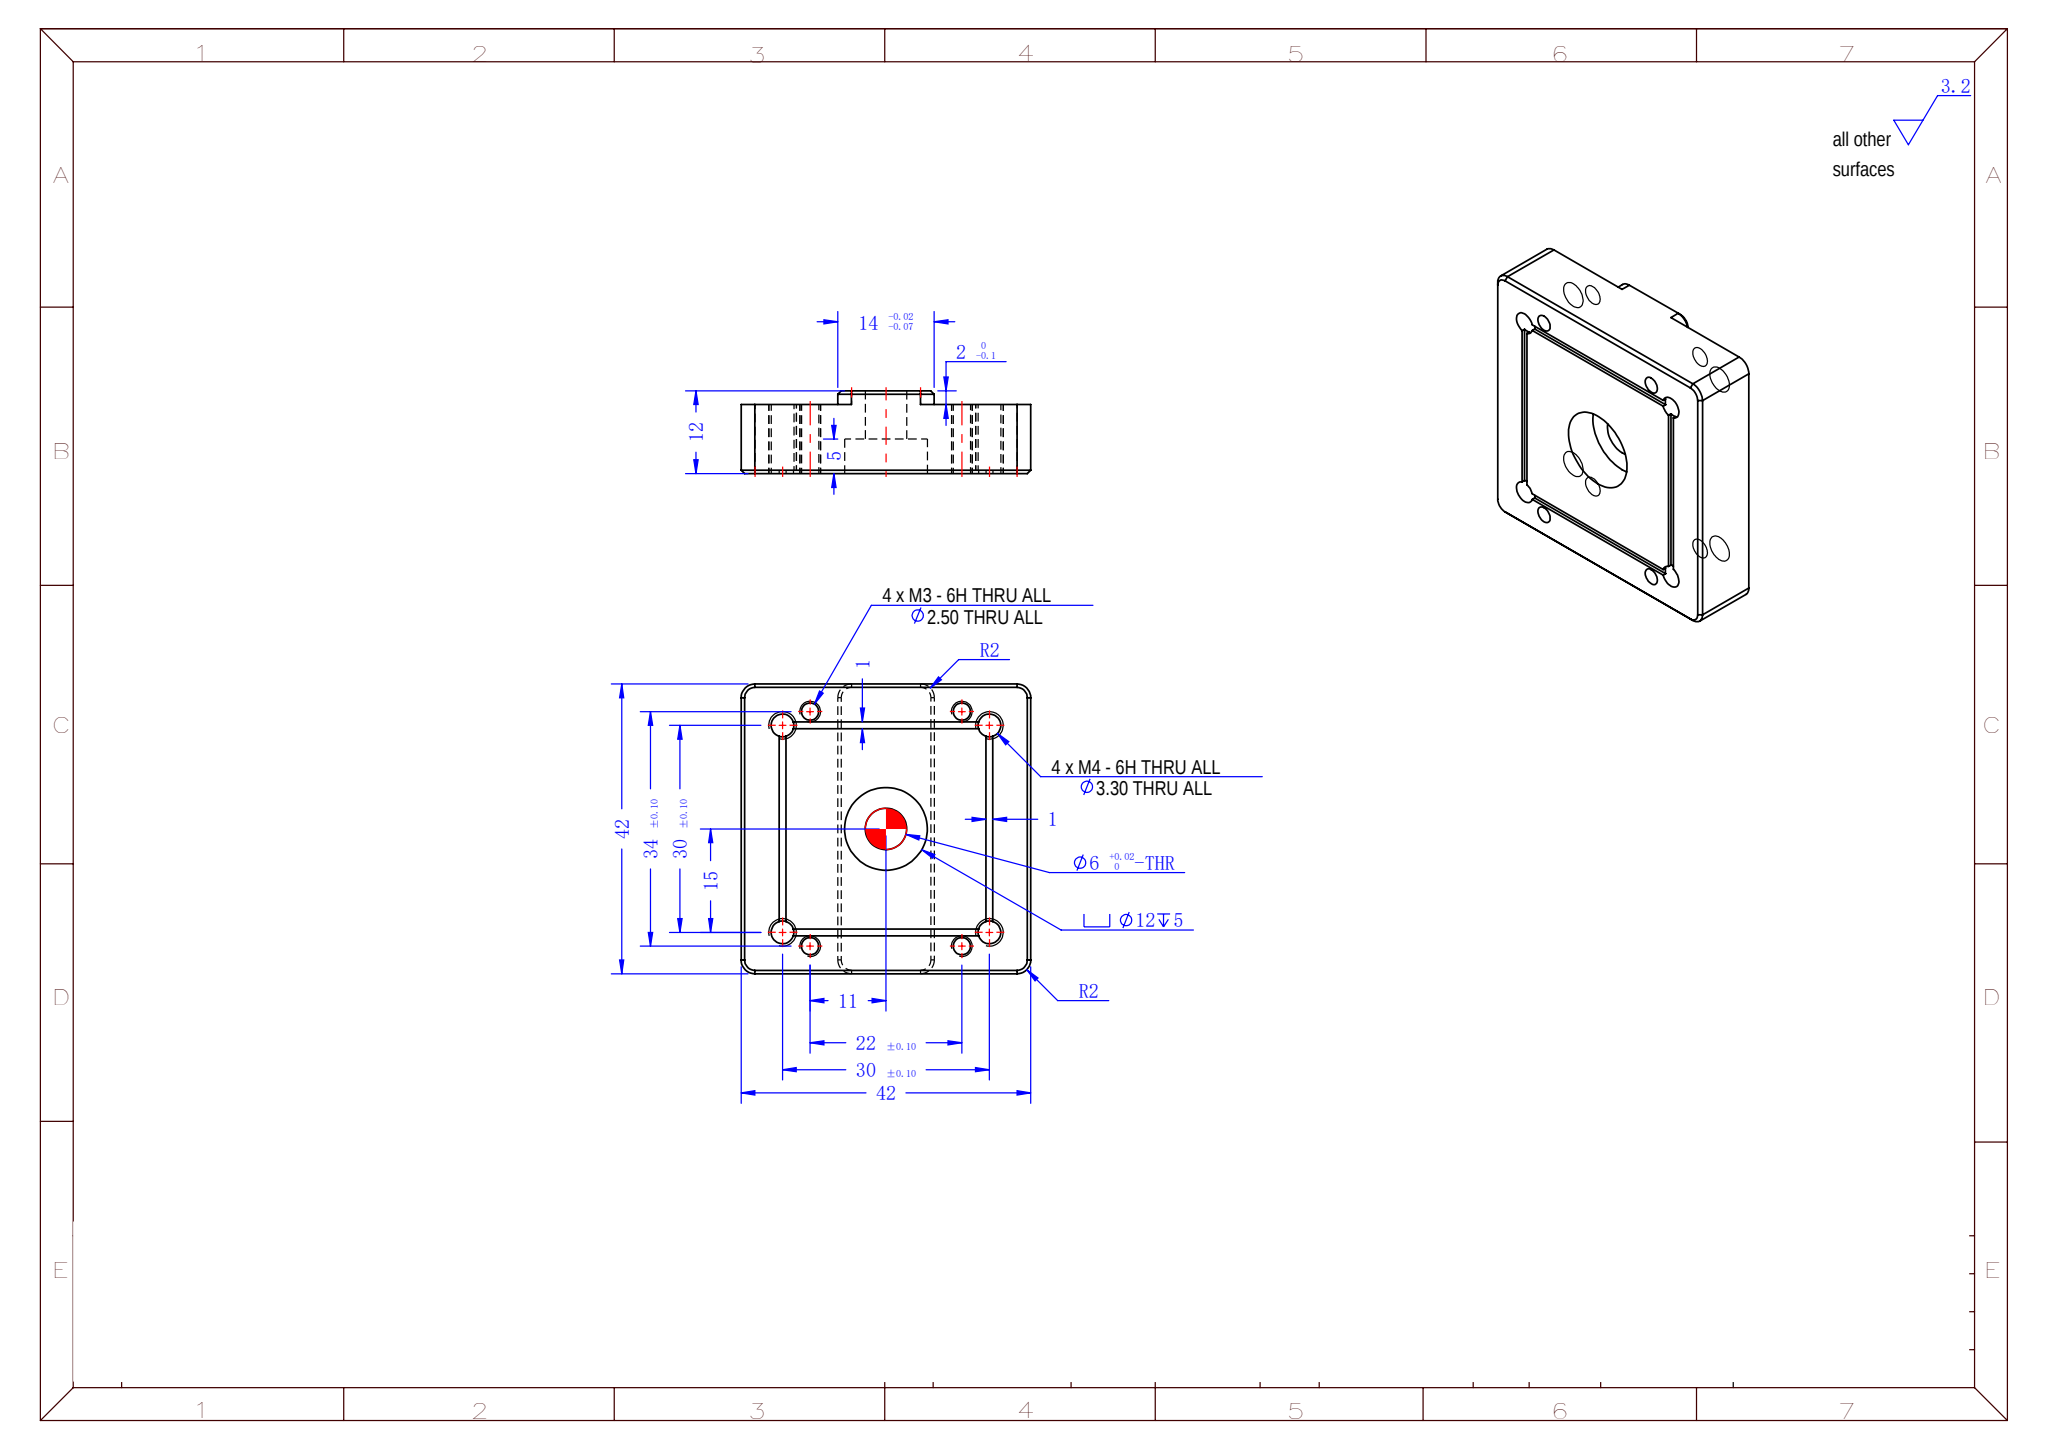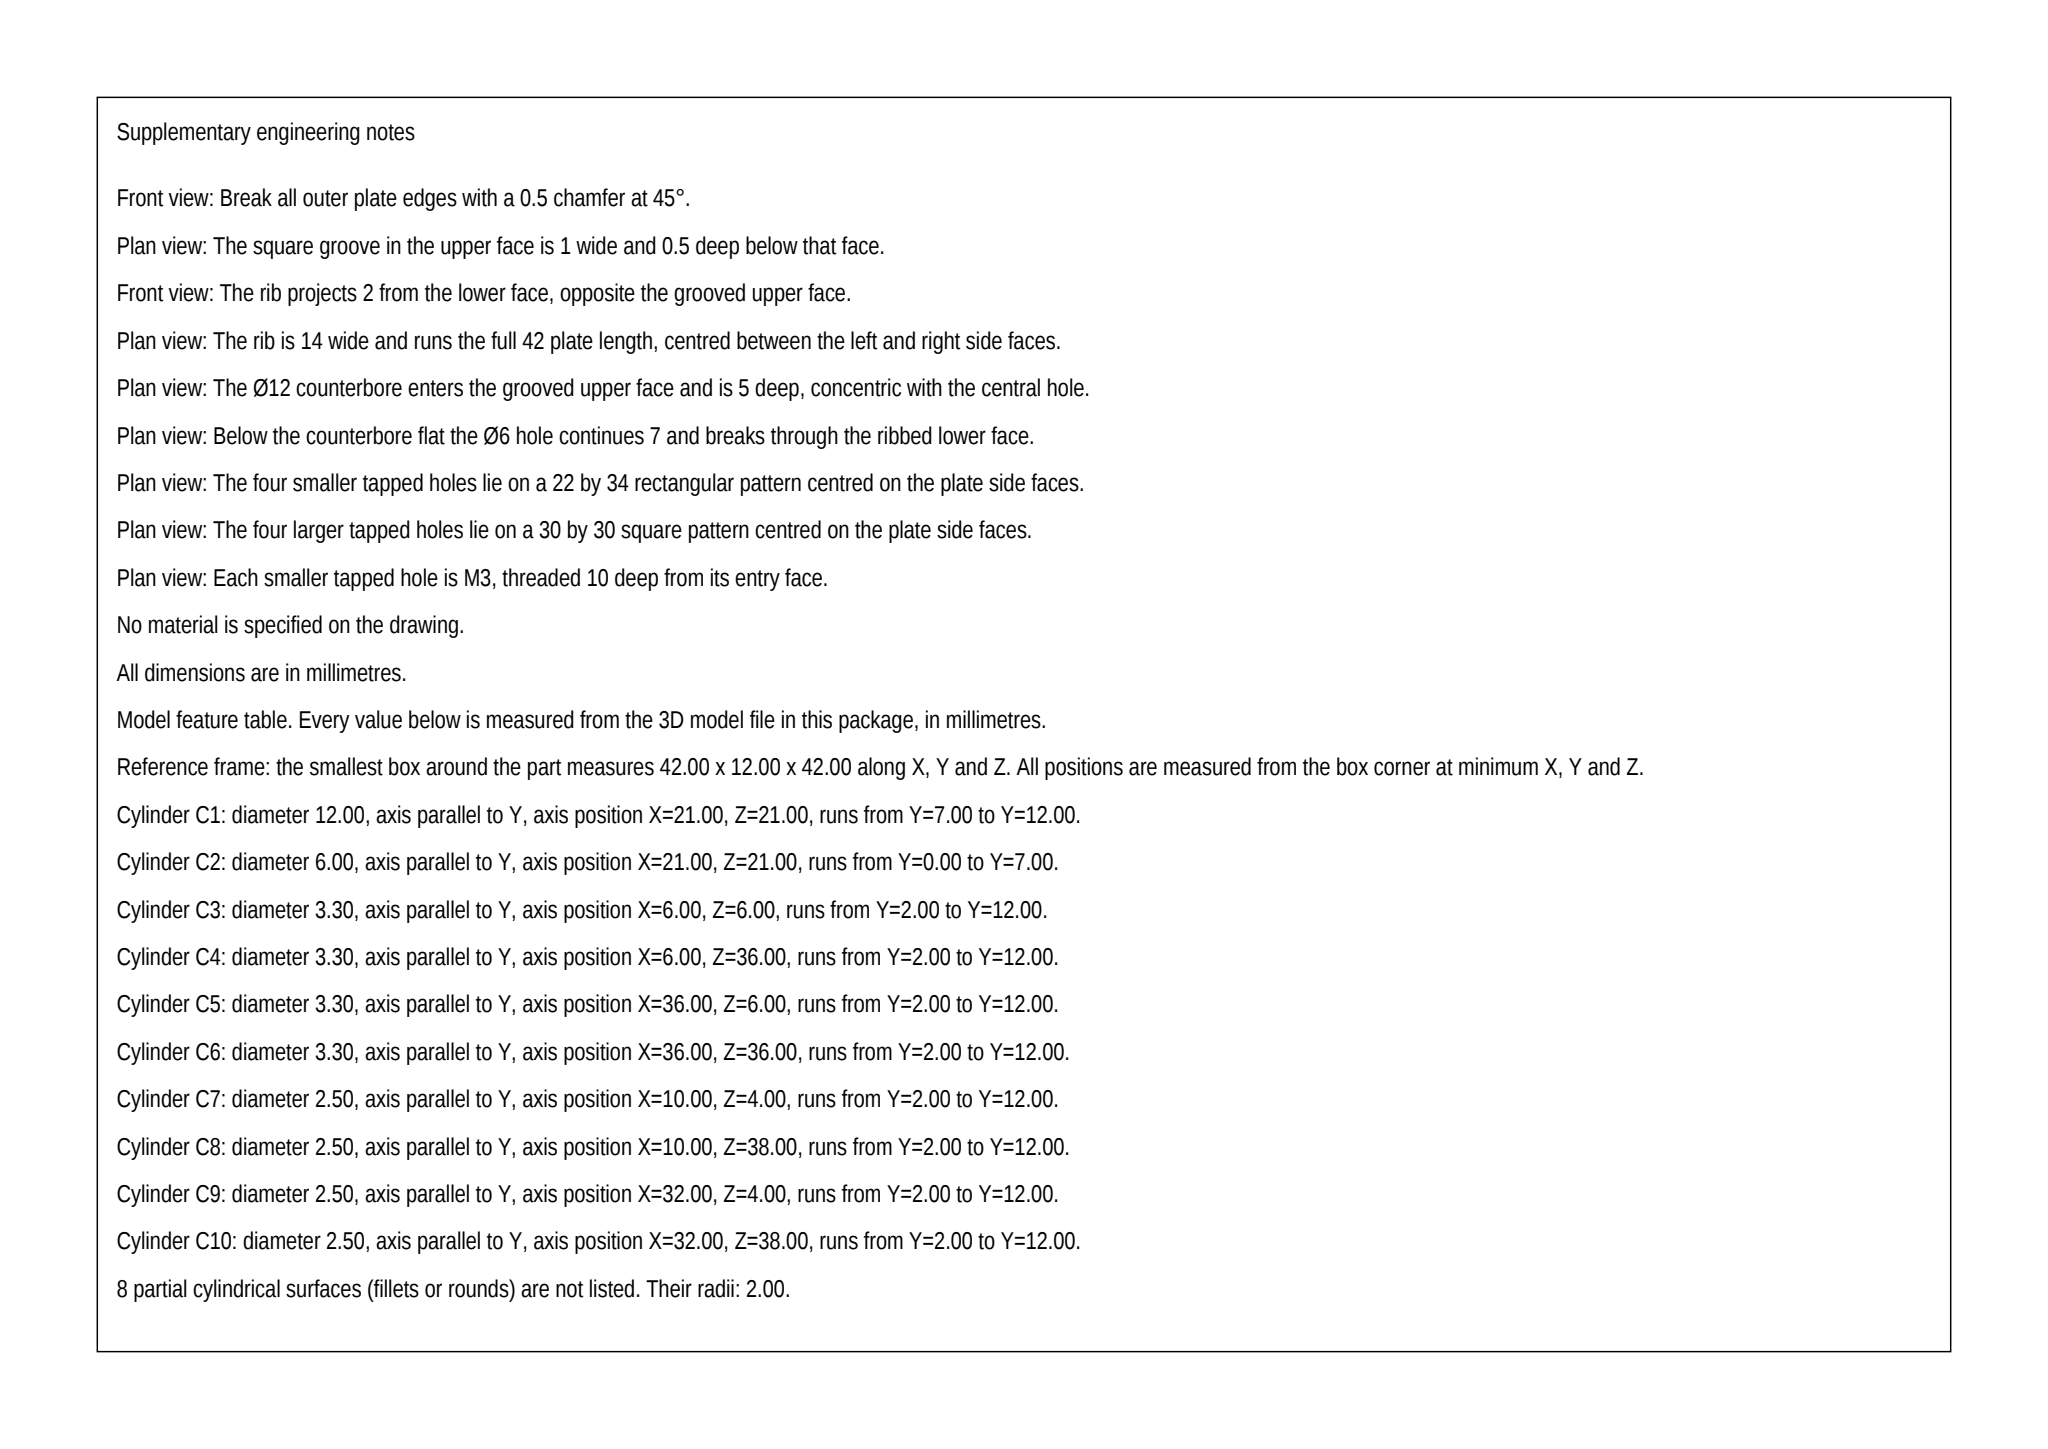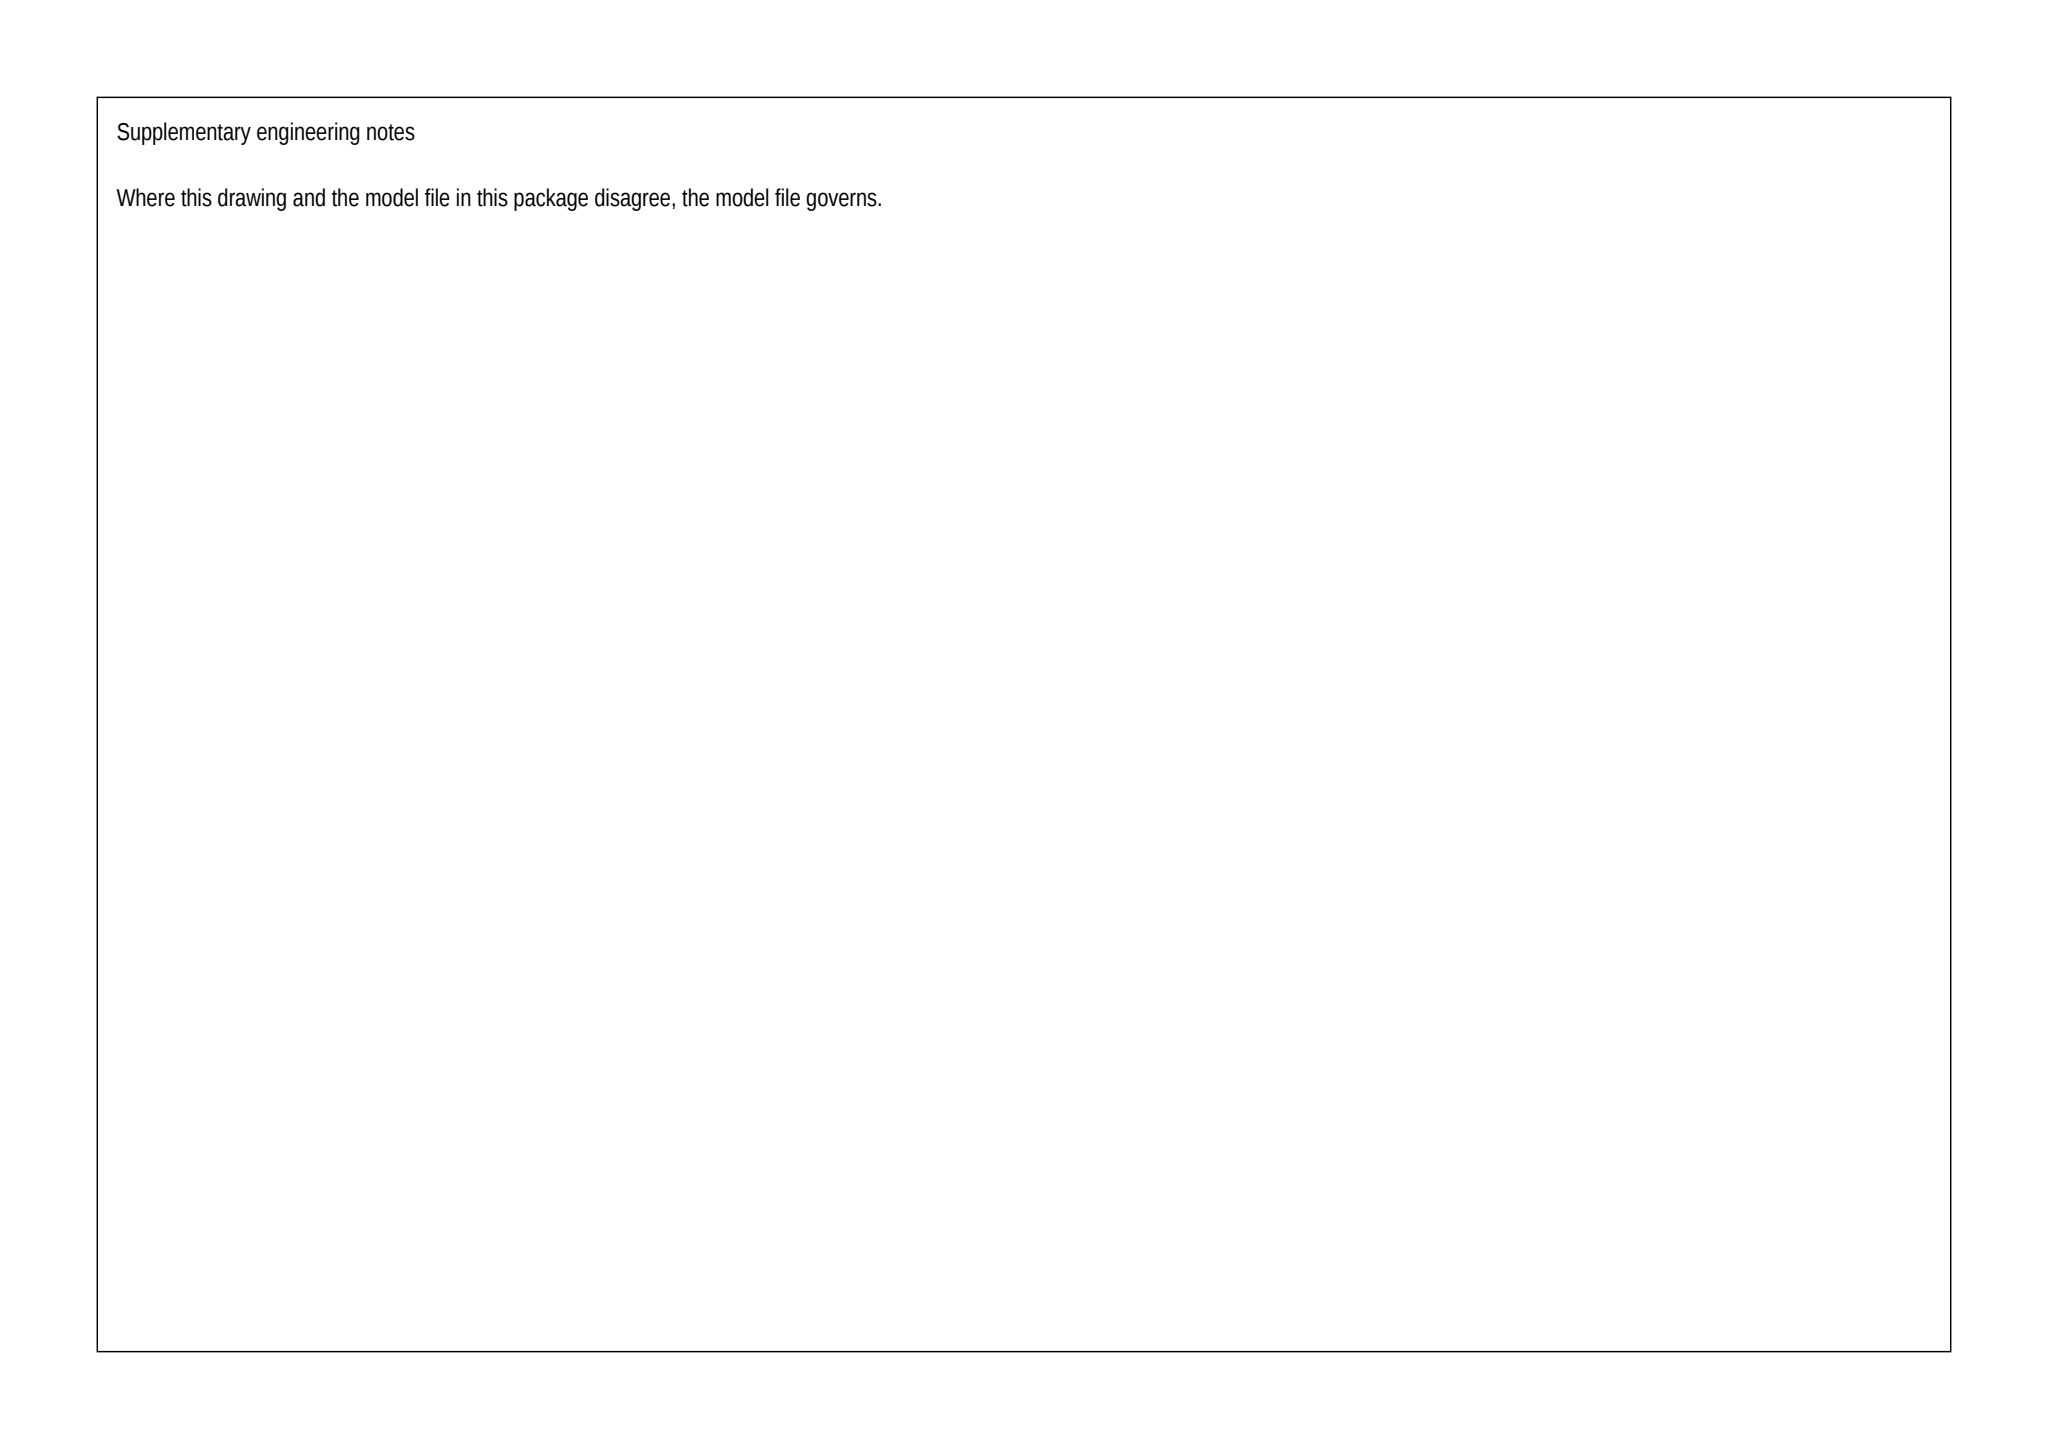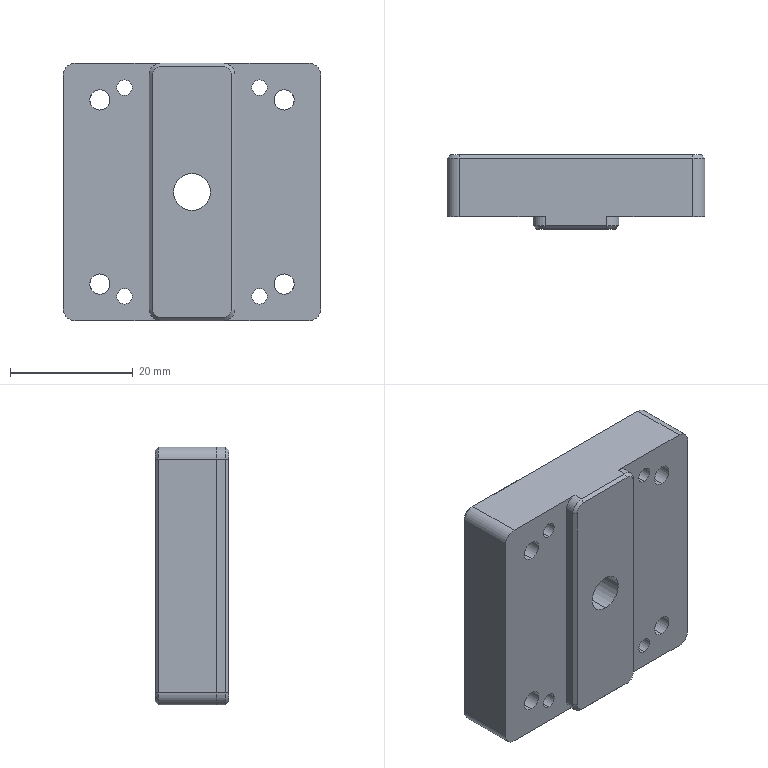Part | SolidWorks | mm | 1 solid | 68 faces | box 42 x 12 x 42 mm | volume 17386 mm3 | plane 32 | cylinder 28 | cone 8 | commonest cylinder face diameters 2.5 x8 3.3 x8 4 x8 6 x2 12 x2
Drawing notes:
4 x M3 THD HOLES: CSK Ø3.0 X 90°, BOTH FACES | from the solid: cones[included_angle,ref_dia]=[90.0,3.0] x8, i.e. 2 per each of 4 Ø2.5 y-axis holes at (10,4),(10,38),(32,4),(32,38)
RING GROOVE ON TOP FACE: 1 WIDE x 0.5 DP | from the solid: y-planes 11.5 vs top face 12.0 -> 0.5 deep; x/z planes 5.5-6.5 & 35.5-36.5 -> 1 wide
GROOVE SIDES 5.5 & 6.5 FROM EACH OUTER EDGE, 4 SIDES | from the solid: axis planes x=5.5/6.5/35.5/36.5 and z=5.5/6.5/35.5/36.5 within 42 x 42 bbox
2x Ø12 DP 5 - BOTH FACES, COAX WITH Ø6 BORE | from the solid: dia 12 cyl, axis y at (21,21), length 5, count 2; Ø6 bore at same axis
build123d program:
from build123d import *

# Parameters (mm, degrees)
SKETCH1_W                 = 42
SKETCH1_H                 = 42
BOSS_EXTRUDE1_DEPTH       = 5
SKETCH2_R                 = 1
CUT_EXTRUDE1_DEPTH        = 32.337
M4_TAPPED_HOLE1_D         = 3.3
SKETCH5_W                 = 14
SKETCH5_H                 = 42
BOSS_EXTRUDE2_DEPTH       = 2
FILLET1_R                 = 2
CHAMFER1_SIZE             = 0.5
SKETCH6_W                 = 31
SKETCH6_H                 = 31
SKETCH6_W_2               = 29
SKETCH6_H_2               = 29
CUT_EXTRUDE_THIN1_DEPTH   = 0.5
M3_TAPPED_HOLE1_D         = 2.5
SKETCH9_R                 = 6
CUT_EXTRUDE3_DEPTH        = 5
SIZE_MM_DOWEL_PIN_HOLE1_D = 6


with BuildPart() as part:
    # Sketch1 → Boss-Extrude1 (new, symmetric)
    with BuildSketch(Plane(origin=(0, 0, 0), x_dir=(1, 0, 0), z_dir=(0, 1, 0))):
        Rectangle(SKETCH1_W, SKETCH1_H)
    extrude(amount=BOSS_EXTRUDE1_DEPTH, both=True)

    # Sketch2 → Cut-Extrude1 (cut, through all)
    with BuildSketch(Plane.XZ.offset(5)):
        with Locations(Location((15, 15, 0), (0, 0, 270))):
            Circle(SKETCH2_R)
        with Locations(Location((15, -15, 0), (0, 0, 270))):
            Circle(SKETCH2_R)
        with Locations(Location((-15, -15, 0), (0, 0, 270))):
            Circle(SKETCH2_R)
        with Locations(Location((-15, 15, 0), (0, 0, 270))):
            Circle(SKETCH2_R)
    extrude(amount=-CUT_EXTRUDE1_DEPTH, mode=Mode.SUBTRACT)

    # M4 Tapped Hole1 (through all)
    with Locations(Plane(origin=(0, -5, 0), x_dir=(-1, 0, 0), z_dir=(0, -1, 0))):
        with Locations((-15, -15), (-15, 15), (15, 15), (15, -15)):
            Hole(M4_TAPPED_HOLE1_D / 2)

    # Sketch5 → Boss-Extrude2 (add)
    with BuildSketch(Plane.XZ.offset(5)):
        Rectangle(SKETCH5_W, SKETCH5_H)
    extrude(amount=BOSS_EXTRUDE2_DEPTH)

    # Fillet1
    fillet1_edges = [part.edges().sort_by_distance(p)[0] for p in [
        (7, -6, -21),
        (7, -6, 21),
        (-7, -6, 21),
        (-7, -6, -21),
        (21, 0, 21),
        (-21, 0, 21),
        (-21, 0, -21),
        (21, 0, -21),
    ]]
    fillet(fillet1_edges, radius=FILLET1_R)

    # Chamfer1
    chamfer1_edges = [part.edges().sort_by_distance(p)[0] for p in [
        (0, -7, -21),
        (0, 5, -21),
        (-7, -7, 0),
        (7, -7, 0),
        (0, -7, 21),
        (-6.414, -7, 20.414),
        (6.414, -7, 20.414),
        (6.414, -7, -20.414),
        (-6.414, -7, -20.414),
        (0, 5, 21),
        (21, 5, 0),
        (-21, 5, 0),
        (-20.414, 5, 20.414),
        (20.414, 5, -20.414),
        (-20.414, 5, -20.414),
        (20.414, 5, 20.414),
    ]]
    chamfer(chamfer1_edges, length=CHAMFER1_SIZE)

    # Sketch6 → Cut-Extrude-Thin1 (cut)
    with BuildSketch(Plane(origin=(0, 5, 0), x_dir=(1, 0, 0), z_dir=(0, 1, 0))):
        Rectangle(SKETCH6_W, SKETCH6_H)
        Rectangle(SKETCH6_W_2, SKETCH6_H_2, mode=Mode.SUBTRACT)
    extrude(amount=-CUT_EXTRUDE_THIN1_DEPTH, mode=Mode.SUBTRACT)

    # M3 Tapped Hole1 (through all)
    with Locations(Plane(origin=(0, -5, 0), x_dir=(-1, 0, 0), z_dir=(0, -1, 0))):
        with Locations((-11, -17), (-11, 17), (11, 17), (11, -17)):
            Hole(M3_TAPPED_HOLE1_D / 2)

    # Sketch9 → Cut-Extrude3 (cut)
    with BuildSketch(Plane(origin=(0, 5, 0), x_dir=(1, 0, 0), z_dir=(0, 1, 0))):
        with Locations(Location((0, 0, 0), (0, 0, 270))):
            Circle(SKETCH9_R)
    extrude(amount=-CUT_EXTRUDE3_DEPTH, mode=Mode.SUBTRACT)

    # Size mm Dowel Pin Hole1 (through all)
    with Locations(Plane(origin=(0, 0, 0), x_dir=(1, 0, 0), z_dir=(0, 1, 0))):
        with Locations((0, 0)):
            Hole(SIZE_MM_DOWEL_PIN_HOLE1_D / 2)


solid = part.part